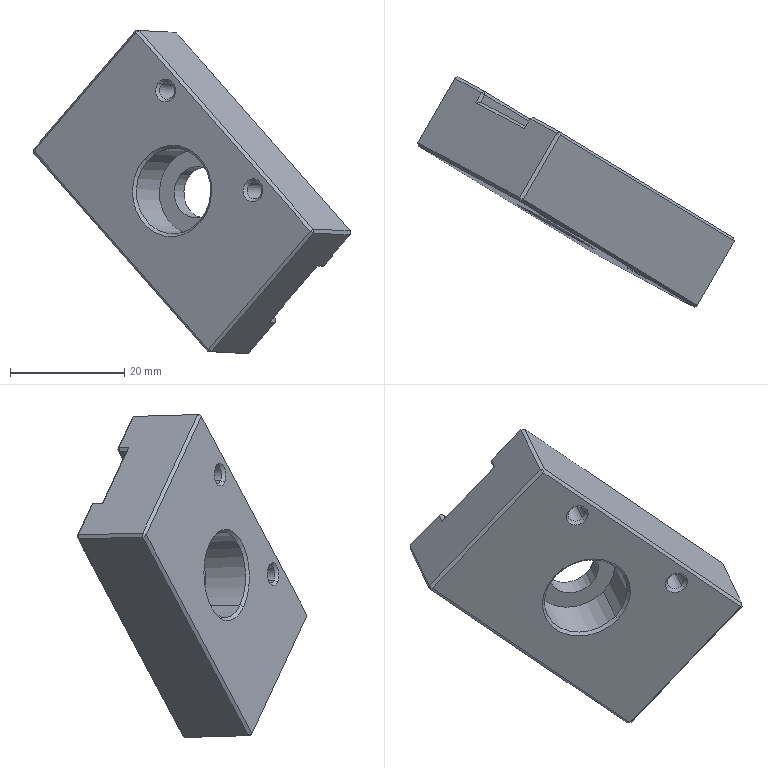Component | SolidWorks | 3z0-123-1 | 1 solid | 63 faces | box 55.38 x 40.27 x 56.56 mm | volume 18030 mm3 | plane 45 | cone 10 | cylinder 8 | commonest cylinder face diameters 3 x4 15 x2 9 x2
build123d program:
from build123d import *

# Parameters (mm, degrees)
SKETCH1_W                                       = 50.8
SKETCH1_H                                       = 30
BOSS_EXTRUDE1_DEPTH                             = 14
M8_HEX_SOCKET_HEAD_CAP_SCREW_CBORE1_D           = 9
M8_HEX_SOCKET_HEAD_CAP_SCREW_CBORE1_CBORE_D     = 15
M8_HEX_SOCKET_HEAD_CAP_SCREW_CBORE1_CBORE_DEPTH = 8.6
SKETCH4_W                                       = 4
SKETCH4_H                                       = 12.8
CUT_EXTRUDE1_DEPTH                              = 55.787
SIZE_MM_DOWEL_PIN_HOLE1_D                       = 3
SIZE_MM_DOWEL_PIN_HOLE1_DEPTH                   = 101.5
SIZE_MM_DOWEL_PIN_HOLE1_TIP                     = 0.9013
CHAMFER1_SIZE                                   = 0.5


with BuildPart() as part:
    # Sketch1 → Boss-Extrude1 (new body)
    with BuildSketch(Plane.XY):
        Rectangle(SKETCH1_W, SKETCH1_H)
    extrude(amount=BOSS_EXTRUDE1_DEPTH)

    # M8 Hex Socket Head Cap Screw CBORE1 (through all)
    with Locations(Plane(origin=(0, 0, 0), x_dir=(-1, 0, 0), z_dir=(0, 0, -1))):
        with Locations((0, 0)):
            CounterBoreHole(M8_HEX_SOCKET_HEAD_CAP_SCREW_CBORE1_D / 2, M8_HEX_SOCKET_HEAD_CAP_SCREW_CBORE1_CBORE_D / 2, M8_HEX_SOCKET_HEAD_CAP_SCREW_CBORE1_CBORE_DEPTH)

    # Sketch4 → Cut-Extrude1 (cut, through all)
    with BuildSketch(Plane.ZY.offset(25.4)):
        with Locations((14, 0)):
            Rectangle(SKETCH4_W, SKETCH4_H)
    extrude(amount=-CUT_EXTRUDE1_DEPTH, mode=Mode.SUBTRACT)

    # Size mm Dowel Pin Hole1
    with Locations(Plane(origin=(-13.4, -11.5, 0), x_dir=(-1, 0, 0), z_dir=(0, 0, -1))):
        with Locations((0, 0), (-25, -0.004294)):
            Hole(SIZE_MM_DOWEL_PIN_HOLE1_D / 2, depth=SIZE_MM_DOWEL_PIN_HOLE1_DEPTH)
            with Locations((0, 0, -(SIZE_MM_DOWEL_PIN_HOLE1_DEPTH + SIZE_MM_DOWEL_PIN_HOLE1_TIP / 2))):  # 118° drill point
                Cone(0, SIZE_MM_DOWEL_PIN_HOLE1_D / 2, SIZE_MM_DOWEL_PIN_HOLE1_TIP, mode=Mode.SUBTRACT)

    # Chamfer1
    chamfer1_edges = [part.edges().sort_by_distance(p)[0] for p in [
        (-25.4, 10.7, 14),
        (0, -15, 14),
        (7.5, 0, 0),
        (25.4, 10.7, 14),
        (-25.4, -10.7, 14),
        (0, -6.4, 14),
        (0, 6.4, 14),
        (25.4, 0, 12),
        (-25.4, 6.4, 13),
        (25.4, -6.4, 13),
        (25.4, 6.4, 13),
        (-25.4, -6.4, 13),
        (-25.4, 0, 12),
        (25.4, -10.7, 14),
        (10.1, -11.504, 14),
        (10.1, -11.504, 0),
        (0, -15, 0),
        (-25.4, 0, 0),
        (-14.9, -11.5, 14),
        (-14.9, -11.5, 0),
        (0, 15, 0),
        (25.4, 0, 0),
        (0, 15, 14),
        (25.4, -15, 7),
        (-25.4, -15, 7),
        (-25.4, 15, 7),
        (25.4, 15, 7),
    ]]
    chamfer(chamfer1_edges, length=CHAMFER1_SIZE)


solid = part.part

# Placed as in the assembly
solid = solid.moved(Location((-76.86, -87.817, 77.38), (-91.664, 29.849, 45.13)))